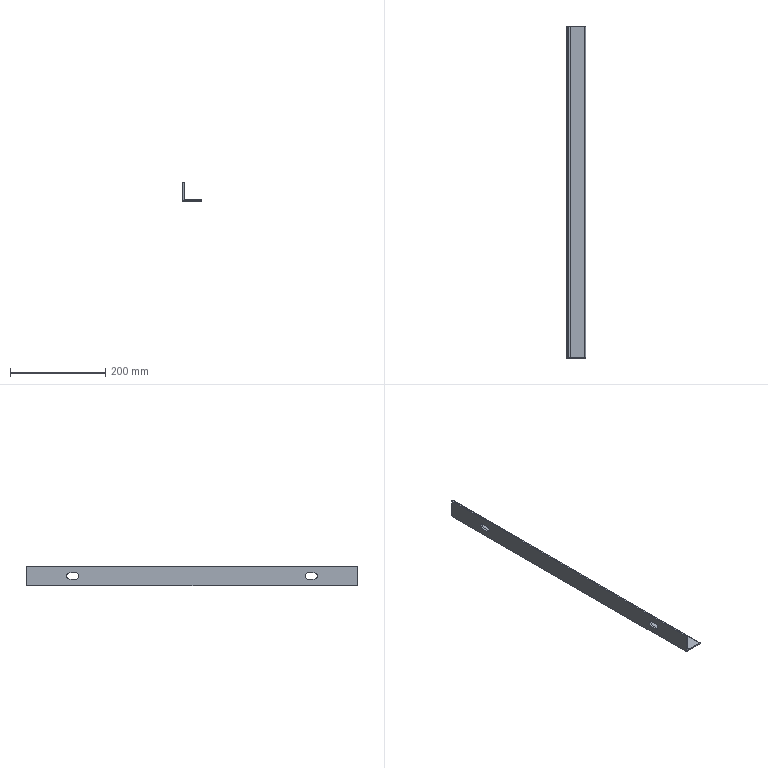Component | SolidWorks | FrameAssembly-1_BeamAngleSteel-1 | 1 solid | 21 faces | box 40 x 696 x 40 mm | volume 210483 mm3 | plane 14 | cylinder 7 | commonest cylinder face diameters 13 x4 2.667 x2 7 x1
build123d program:
from build123d import *

# Parameters (mm, degrees)
BASE_DEPTH         = 696
CUT_EXTRUDE1_DEPTH = 5
CHAMFER1_SIZE      = 1.5


with BuildPart() as part:
    # Sketch1 → Base (new body)
    with BuildSketch(Plane.YZ):
        with BuildLine():
            Line((0, 40), (0, 0))
            Line((0, 0), (40, 0))
            Line((40, 0), (40, 2.667))
            ThreePointArc((40, 2.667), (39.609, 3.609), (38.667, 4))
            Line((38.667, 4), (7.5, 4))
            ThreePointArc((7.5, 4), (5.025, 5.025), (4, 7.5))
            Line((4, 7.5), (4, 38.667))
            ThreePointArc((4, 38.667), (3.609, 39.609), (2.667, 40))
            Line((2.667, 40), (0, 40))
        make_face()
    extrude(amount=BASE_DEPTH)

    # Sketch1_2 → Cut-Extrude1 (cut)
    with BuildSketch(Plane(origin=(0, 4, 0), x_dir=(-1, 0, 0), z_dir=(0, 1, 0))):
        with BuildLine():
            Line((-92, 13.5), (-104, 13.5))
            ThreePointArc((-104, 13.5), (-110.5, 20), (-104, 26.5))
            Line((-104, 26.5), (-92, 26.5))
            ThreePointArc((-92, 26.5), (-85.5, 20), (-92, 13.5))
        make_face()
        with BuildLine():
            Line((-592, 13.5), (-604, 13.5))
            ThreePointArc((-604, 13.5), (-610.5, 20), (-604, 26.5))
            Line((-604, 26.5), (-592, 26.5))
            ThreePointArc((-592, 26.5), (-585.5, 20), (-592, 13.5))
        make_face()
    extrude(amount=-CUT_EXTRUDE1_DEPTH, mode=Mode.SUBTRACT)

    # Chamfer1
    chamfer1_edges = [part.edges().sort_by_distance(p)[0] for p in [
        (696, 20, 0),
        (0, 20, 0),
    ]]
    chamfer(chamfer1_edges, length=CHAMFER1_SIZE)


solid = part.part

# Placed as in the assembly
solid = solid.moved(Location((-927.848, 492.395, 0), (0, 0, -90)))
STEP:
#1=COLOUR_RGB('',0.7922,0.8196,0.9333);
#2=FILL_AREA_STYLE_COLOUR('',#1);
#3=FILL_AREA_STYLE('',(#2));
#4=SURFACE_STYLE_FILL_AREA(#3);
#5=SURFACE_SIDE_STYLE('',(#4));
#6=SURFACE_STYLE_USAGE(.BOTH.,#5);
#7=PRESENTATION_STYLE_ASSIGNMENT((#6));
#8=CARTESIAN_POINT('',(-36.424,19.386,1.575));
#9=VERTEX_POINT('',#8);
#10=CARTESIAN_POINT('',(-36.529,19.386,1.575));
#11=VERTEX_POINT('',#10);
#12=CARTESIAN_POINT('',(-36.529,19.386,1.575));
#13=DIRECTION('',(-1.,0.,0.));
#14=VECTOR('',#13,39.37);
#15=LINE('',#12,#14);
#16=EDGE_CURVE('',#9,#11,#15,.T.);
#17=ORIENTED_EDGE('',*,*,#16,.T.);
#18=CARTESIAN_POINT('',(-36.529,-8.016,1.575));
#19=VERTEX_POINT('',#18);
#20=CARTESIAN_POINT('',(-36.529,-8.016,1.575));
#21=DIRECTION('',(0.,1.,0.));
#22=VECTOR('',#21,39.37);
#23=LINE('',#20,#22);
#24=EDGE_CURVE('',#19,#11,#23,.T.);
#25=ORIENTED_EDGE('',*,*,#24,.F.);
#26=CARTESIAN_POINT('',(-36.424,-8.016,1.575));
#27=VERTEX_POINT('',#26);
#28=CARTESIAN_POINT('',(-36.529,-8.016,1.575));
#29=DIRECTION('',(-1.,0.,0.));
#30=VECTOR('',#29,39.37);
#31=LINE('',#28,#30);
#32=EDGE_CURVE('',#27,#19,#31,.T.);
#33=ORIENTED_EDGE('',*,*,#32,.F.);
#34=CARTESIAN_POINT('',(-36.424,-8.016,1.575));
#35=DIRECTION('',(0.,1.,0.));
#36=VECTOR('',#35,39.37);
#37=LINE('',#34,#36);
#38=EDGE_CURVE('',#27,#9,#37,.T.);
#39=ORIENTED_EDGE('',*,*,#38,.T.);
#40=EDGE_LOOP('',(#17,#25,#33,#39));
#41=FACE_OUTER_BOUND('',#40,.T.);
#42=CARTESIAN_POINT('',(-36.529,-8.016,1.575));
#43=DIRECTION('',(-0.,0.,-1.));
#44=DIRECTION('',(0.,1.,0.));
#45=AXIS2_PLACEMENT_3D('',#42,#43,#44);
#46=PLANE('',#45);
#47=ADVANCED_FACE('',(#41),#46,.F.);
#48=CARTESIAN_POINT('',(-36.529,-4.394,0.5315));
#49=VERTEX_POINT('',#48);
#50=CARTESIAN_POINT('',(-36.529,-3.921,0.5315));
#51=VERTEX_POINT('',#50);
#52=CARTESIAN_POINT('',(-36.529,-8.016,0.5315));
#53=DIRECTION('',(0.,1.,0.));
#54=VECTOR('',#53,39.37);
#55=LINE('',#52,#54);
#56=EDGE_CURVE('',#49,#51,#55,.T.);
#57=ORIENTED_EDGE('',*,*,#56,.T.);
#58=CARTESIAN_POINT('',(-36.529,-3.921,1.043));
#59=VERTEX_POINT('',#58);
#60=CARTESIAN_POINT('',(-36.529,-3.921,0.7874));
#61=DIRECTION('',(1.,-0.,-0.));
#62=DIRECTION('',(0.,-0.,1.));
#63=AXIS2_PLACEMENT_3D('',#60,#61,#62);
#64=CIRCLE('',#63,0.2559);
#65=EDGE_CURVE('',#51,#59,#64,.T.);
#66=ORIENTED_EDGE('',*,*,#65,.T.);
#67=CARTESIAN_POINT('',(-36.529,-4.394,1.043));
#68=VERTEX_POINT('',#67);
#69=CARTESIAN_POINT('',(-36.529,-8.016,1.043));
#70=DIRECTION('',(-0.,-1.,-0.));
#71=VECTOR('',#70,39.37);
#72=LINE('',#69,#71);
#73=EDGE_CURVE('',#59,#68,#72,.T.);
#74=ORIENTED_EDGE('',*,*,#73,.T.);
#75=CARTESIAN_POINT('',(-36.529,-4.394,0.7874));
#76=DIRECTION('',(1.,-0.,-0.));
#77=DIRECTION('',(0.,-0.,1.));
#78=AXIS2_PLACEMENT_3D('',#75,#76,#77);
#79=CIRCLE('',#78,0.2559);
#80=EDGE_CURVE('',#68,#49,#79,.T.);
#81=ORIENTED_EDGE('',*,*,#80,.T.);
#82=EDGE_LOOP('',(#57,#66,#74,#81));
#83=FACE_BOUND('',#82,.T.);
#84=CARTESIAN_POINT('',(-36.529,15.291,0.5315));
#85=VERTEX_POINT('',#84);
#86=CARTESIAN_POINT('',(-36.529,15.764,0.5315));
#87=VERTEX_POINT('',#86);
#88=CARTESIAN_POINT('',(-36.529,-8.016,0.5315));
#89=DIRECTION('',(0.,1.,0.));
#90=VECTOR('',#89,39.37);
#91=LINE('',#88,#90);
#92=EDGE_CURVE('',#85,#87,#91,.T.);
#93=ORIENTED_EDGE('',*,*,#92,.T.);
#94=CARTESIAN_POINT('',(-36.529,15.764,1.043));
#95=VERTEX_POINT('',#94);
#96=CARTESIAN_POINT('',(-36.529,15.764,0.7874));
#97=DIRECTION('',(1.,-0.,-0.));
#98=DIRECTION('',(0.,-0.,1.));
#99=AXIS2_PLACEMENT_3D('',#96,#97,#98);
#100=CIRCLE('',#99,0.2559);
#101=EDGE_CURVE('',#87,#95,#100,.T.);
#102=ORIENTED_EDGE('',*,*,#101,.T.);
#103=CARTESIAN_POINT('',(-36.529,15.291,1.043));
#104=VERTEX_POINT('',#103);
#105=CARTESIAN_POINT('',(-36.529,-8.016,1.043));
#106=DIRECTION('',(-0.,-1.,-0.));
#107=VECTOR('',#106,39.37);
#108=LINE('',#105,#107);
#109=EDGE_CURVE('',#95,#104,#108,.T.);
#110=ORIENTED_EDGE('',*,*,#109,.T.);
#111=CARTESIAN_POINT('',(-36.529,15.291,0.7874));
#112=DIRECTION('',(1.,-0.,-0.));
#113=DIRECTION('',(0.,-0.,1.));
#114=AXIS2_PLACEMENT_3D('',#111,#112,#113);
#115=CIRCLE('',#114,0.2559);
#116=EDGE_CURVE('',#104,#85,#115,.T.);
#117=ORIENTED_EDGE('',*,*,#116,.T.);
#118=EDGE_LOOP('',(#93,#102,#110,#117));
#119=FACE_BOUND('',#118,.T.);
#120=CARTESIAN_POINT('',(-36.529,19.386,0.05906));
#121=VERTEX_POINT('',#120);
#122=CARTESIAN_POINT('',(-36.529,19.386,1.575));
#123=DIRECTION('',(-0.,0.,-1.));
#124=VECTOR('',#123,39.37);
#125=LINE('',#122,#124);
#126=EDGE_CURVE('',#11,#121,#125,.T.);
#127=ORIENTED_EDGE('',*,*,#126,.T.);
#128=CARTESIAN_POINT('',(-36.529,19.327,-0.));
#129=VERTEX_POINT('',#128);
#130=CARTESIAN_POINT('',(-36.529,19.327,-0.));
#131=DIRECTION('',(-0.,-0.7071,-0.7071));
#132=VECTOR('',#131,39.37);
#133=LINE('',#130,#132);
#134=EDGE_CURVE('',#121,#129,#133,.T.);
#135=ORIENTED_EDGE('',*,*,#134,.T.);
#136=CARTESIAN_POINT('',(-36.529,-7.957,-0.));
#137=VERTEX_POINT('',#136);
#138=CARTESIAN_POINT('',(-36.529,-8.016,-0.));
#139=DIRECTION('',(0.,1.,0.));
#140=VECTOR('',#139,39.37);
#141=LINE('',#138,#140);
#142=EDGE_CURVE('',#137,#129,#141,.T.);
#143=ORIENTED_EDGE('',*,*,#142,.F.);
#144=CARTESIAN_POINT('',(-36.529,-8.016,0.05906));
#145=VERTEX_POINT('',#144);
#146=CARTESIAN_POINT('',(-36.529,-8.016,0.05906));
#147=DIRECTION('',(-0.,-0.7071,0.7071));
#148=VECTOR('',#147,39.37);
#149=LINE('',#146,#148);
#150=EDGE_CURVE('',#137,#145,#149,.T.);
#151=ORIENTED_EDGE('',*,*,#150,.T.);
#152=CARTESIAN_POINT('',(-36.529,-8.016,1.575));
#153=DIRECTION('',(-0.,0.,-1.));
#154=VECTOR('',#153,39.37);
#155=LINE('',#152,#154);
#156=EDGE_CURVE('',#19,#145,#155,.T.);
#157=ORIENTED_EDGE('',*,*,#156,.F.);
#158=ORIENTED_EDGE('',*,*,#24,.T.);
#159=EDGE_LOOP('',(#127,#135,#143,#151,#157,#158));
#160=FACE_OUTER_BOUND('',#159,.T.);
#161=CARTESIAN_POINT('',(-36.529,-8.016,1.575));
#162=DIRECTION('',(1.,-0.,-0.));
#163=DIRECTION('',(0.,-0.,1.));
#164=AXIS2_PLACEMENT_3D('',#161,#162,#163);
#165=PLANE('',#164);
#166=ADVANCED_FACE('',(#83,#119,#160),#165,.F.);
#167=ORIENTED_EDGE('',*,*,#142,.T.);
#168=CARTESIAN_POINT('',(-34.955,19.327,-0.));
#169=VERTEX_POINT('',#168);
#170=CARTESIAN_POINT('',(-34.955,19.327,-0.));
#171=DIRECTION('',(1.,-0.,-0.));
#172=VECTOR('',#171,39.37);
#173=LINE('',#170,#172);
#174=EDGE_CURVE('',#129,#169,#173,.T.);
#175=ORIENTED_EDGE('',*,*,#174,.T.);
#176=CARTESIAN_POINT('',(-34.955,-7.957,-0.));
#177=VERTEX_POINT('',#176);
#178=CARTESIAN_POINT('',(-34.955,-8.016,-0.));
#179=DIRECTION('',(0.,1.,0.));
#180=VECTOR('',#179,39.37);
#181=LINE('',#178,#180);
#182=EDGE_CURVE('',#177,#169,#181,.T.);
#183=ORIENTED_EDGE('',*,*,#182,.F.);
#184=CARTESIAN_POINT('',(-36.529,-7.957,-0.));
#185=DIRECTION('',(-1.,0.,0.));
#186=VECTOR('',#185,39.37);
#187=LINE('',#184,#186);
#188=EDGE_CURVE('',#177,#137,#187,.T.);
#189=ORIENTED_EDGE('',*,*,#188,.T.);
#190=EDGE_LOOP('',(#167,#175,#183,#189));
#191=FACE_OUTER_BOUND('',#190,.T.);
#192=CARTESIAN_POINT('',(-36.529,-8.016,-0.));
#193=DIRECTION('',(0.,-0.,1.));
#194=DIRECTION('',(-0.,-1.,-0.));
#195=AXIS2_PLACEMENT_3D('',#192,#193,#194);
#196=PLANE('',#195);
#197=ADVANCED_FACE('',(#191),#196,.F.);
#198=ORIENTED_EDGE('',*,*,#182,.T.);
#199=CARTESIAN_POINT('',(-34.955,19.386,0.05906));
#200=VERTEX_POINT('',#199);
#201=CARTESIAN_POINT('',(-34.955,19.327,-0.));
#202=DIRECTION('',(0.,0.7071,0.7071));
#203=VECTOR('',#202,39.37);
#204=LINE('',#201,#203);
#205=EDGE_CURVE('',#169,#200,#204,.T.);
#206=ORIENTED_EDGE('',*,*,#205,.T.);
#207=CARTESIAN_POINT('',(-34.955,19.386,0.105));
#208=VERTEX_POINT('',#207);
#209=CARTESIAN_POINT('',(-34.955,19.386,-0.));
#210=DIRECTION('',(0.,-0.,1.));
#211=VECTOR('',#210,39.37);
#212=LINE('',#209,#211);
#213=EDGE_CURVE('',#200,#208,#212,.T.);
#214=ORIENTED_EDGE('',*,*,#213,.T.);
#215=CARTESIAN_POINT('',(-34.955,-8.016,0.105));
#216=VERTEX_POINT('',#215);
#217=CARTESIAN_POINT('',(-34.955,-8.016,0.105));
#218=DIRECTION('',(0.,1.,0.));
#219=VECTOR('',#218,39.37);
#220=LINE('',#217,#219);
#221=EDGE_CURVE('',#216,#208,#220,.T.);
#222=ORIENTED_EDGE('',*,*,#221,.F.);
#223=CARTESIAN_POINT('',(-34.955,-8.016,0.05906));
#224=VERTEX_POINT('',#223);
#225=CARTESIAN_POINT('',(-34.955,-8.016,-0.));
#226=DIRECTION('',(0.,-0.,1.));
#227=VECTOR('',#226,39.37);
#228=LINE('',#225,#227);
#229=EDGE_CURVE('',#224,#216,#228,.T.);
#230=ORIENTED_EDGE('',*,*,#229,.F.);
#231=CARTESIAN_POINT('',(-34.955,-8.016,0.05906));
#232=DIRECTION('',(0.,0.7071,-0.7071));
#233=VECTOR('',#232,39.37);
#234=LINE('',#231,#233);
#235=EDGE_CURVE('',#224,#177,#234,.T.);
#236=ORIENTED_EDGE('',*,*,#235,.T.);
#237=EDGE_LOOP('',(#198,#206,#214,#222,#230,#236));
#238=FACE_OUTER_BOUND('',#237,.T.);
#239=CARTESIAN_POINT('',(-34.955,-8.016,-0.));
#240=DIRECTION('',(-1.,0.,0.));
#241=DIRECTION('',(-0.,0.,-1.));
#242=AXIS2_PLACEMENT_3D('',#239,#240,#241);
#243=PLANE('',#242);
#244=ADVANCED_FACE('',(#238),#243,.F.);
#245=CARTESIAN_POINT('',(-35.007,19.386,0.1575));
#246=VERTEX_POINT('',#245);
#247=CARTESIAN_POINT('',(-35.007,19.386,0.105));
#248=DIRECTION('',(-0.,-1.,-0.));
#249=DIRECTION('',(0.,0.,-1.));
#250=AXIS2_PLACEMENT_3D('',#247,#248,#249);
#251=CIRCLE('',#250,0.05249);
#252=EDGE_CURVE('',#208,#246,#251,.T.);
#253=ORIENTED_EDGE('',*,*,#252,.T.);
#254=CARTESIAN_POINT('',(-35.007,-8.016,0.1575));
#255=VERTEX_POINT('',#254);
#256=CARTESIAN_POINT('',(-35.007,-8.016,0.1575));
#257=DIRECTION('',(0.,1.,0.));
#258=VECTOR('',#257,39.37);
#259=LINE('',#256,#258);
#260=EDGE_CURVE('',#255,#246,#259,.T.);
#261=ORIENTED_EDGE('',*,*,#260,.F.);
#262=CARTESIAN_POINT('',(-35.007,-8.016,0.105));
#263=DIRECTION('',(-0.,-1.,-0.));
#264=DIRECTION('',(0.,0.,-1.));
#265=AXIS2_PLACEMENT_3D('',#262,#263,#264);
#266=CIRCLE('',#265,0.05249);
#267=EDGE_CURVE('',#216,#255,#266,.T.);
#268=ORIENTED_EDGE('',*,*,#267,.F.);
#269=ORIENTED_EDGE('',*,*,#221,.T.);
#270=EDGE_LOOP('',(#253,#261,#268,#269));
#271=FACE_OUTER_BOUND('',#270,.T.);
#272=CARTESIAN_POINT('',(-35.007,-8.016,0.105));
#273=DIRECTION('',(0.,1.,0.));
#274=DIRECTION('',(0.,-0.,1.));
#275=AXIS2_PLACEMENT_3D('',#272,#273,#274);
#276=CYLINDRICAL_SURFACE('',#275,0.05249);
#277=ADVANCED_FACE('',(#271),#276,.T.);
#278=CARTESIAN_POINT('',(-36.234,19.386,0.1575));
#279=VERTEX_POINT('',#278);
#280=CARTESIAN_POINT('',(-36.234,19.386,0.1575));
#281=DIRECTION('',(-1.,0.,0.));
#282=VECTOR('',#281,39.37);
#283=LINE('',#280,#282);
#284=EDGE_CURVE('',#246,#279,#283,.T.);
#285=ORIENTED_EDGE('',*,*,#284,.T.);
#286=CARTESIAN_POINT('',(-36.234,-8.016,0.1575));
#287=VERTEX_POINT('',#286);
#288=CARTESIAN_POINT('',(-36.234,-8.016,0.1575));
#289=DIRECTION('',(0.,1.,0.));
#290=VECTOR('',#289,39.37);
#291=LINE('',#288,#290);
#292=EDGE_CURVE('',#287,#279,#291,.T.);
#293=ORIENTED_EDGE('',*,*,#292,.F.);
#294=CARTESIAN_POINT('',(-36.234,-8.016,0.1575));
#295=DIRECTION('',(-1.,0.,0.));
#296=VECTOR('',#295,39.37);
#297=LINE('',#294,#296);
#298=EDGE_CURVE('',#255,#287,#297,.T.);
#299=ORIENTED_EDGE('',*,*,#298,.F.);
#300=ORIENTED_EDGE('',*,*,#260,.T.);
#301=EDGE_LOOP('',(#285,#293,#299,#300));
#302=FACE_OUTER_BOUND('',#301,.T.);
#303=CARTESIAN_POINT('',(-36.234,-8.016,0.1575));
#304=DIRECTION('',(-0.,0.,-1.));
#305=DIRECTION('',(0.,1.,0.));
#306=AXIS2_PLACEMENT_3D('',#303,#304,#305);
#307=PLANE('',#306);
#308=ADVANCED_FACE('',(#302),#307,.F.);
#309=CARTESIAN_POINT('',(-36.372,19.386,0.2953));
#310=VERTEX_POINT('',#309);
#311=CARTESIAN_POINT('',(-36.234,19.386,0.2953));
#312=DIRECTION('',(0.,1.,0.));
#313=DIRECTION('',(0.,0.,-1.));
#314=AXIS2_PLACEMENT_3D('',#311,#312,#313);
#315=CIRCLE('',#314,0.1378);
#316=EDGE_CURVE('',#279,#310,#315,.T.);
#317=ORIENTED_EDGE('',*,*,#316,.T.);
#318=CARTESIAN_POINT('',(-36.372,-8.016,0.2953));
#319=VERTEX_POINT('',#318);
#320=CARTESIAN_POINT('',(-36.372,-8.016,0.2953));
#321=DIRECTION('',(0.,1.,0.));
#322=VECTOR('',#321,39.37);
#323=LINE('',#320,#322);
#324=EDGE_CURVE('',#319,#310,#323,.T.);
#325=ORIENTED_EDGE('',*,*,#324,.F.);
#326=CARTESIAN_POINT('',(-36.234,-8.016,0.2953));
#327=DIRECTION('',(0.,1.,0.));
#328=DIRECTION('',(0.,0.,-1.));
#329=AXIS2_PLACEMENT_3D('',#326,#327,#328);
#330=CIRCLE('',#329,0.1378);
#331=EDGE_CURVE('',#287,#319,#330,.T.);
#332=ORIENTED_EDGE('',*,*,#331,.F.);
#333=ORIENTED_EDGE('',*,*,#292,.T.);
#334=EDGE_LOOP('',(#317,#325,#332,#333));
#335=FACE_OUTER_BOUND('',#334,.T.);
#336=CARTESIAN_POINT('',(-36.234,-8.016,0.2953));
#337=DIRECTION('',(0.,1.,0.));
#338=DIRECTION('',(0.,-0.,1.));
#339=AXIS2_PLACEMENT_3D('',#336,#337,#338);
#340=CYLINDRICAL_SURFACE('',#339,0.1378);
#341=ADVANCED_FACE('',(#335),#340,.F.);
#342=CARTESIAN_POINT('',(-36.372,-3.921,1.043));
#343=VERTEX_POINT('',#342);
#344=CARTESIAN_POINT('',(-36.372,-4.394,1.043));
#345=VERTEX_POINT('',#344);
#346=CARTESIAN_POINT('',(-36.372,-3.921,1.043));
#347=DIRECTION('',(-0.,-1.,-0.));
#348=VECTOR('',#347,39.37);
#349=LINE('',#346,#348);
#350=EDGE_CURVE('',#343,#345,#349,.T.);
#351=ORIENTED_EDGE('',*,*,#350,.F.);
#352=CARTESIAN_POINT('',(-36.372,-3.921,0.5315));
#353=VERTEX_POINT('',#352);
#354=CARTESIAN_POINT('',(-36.372,-3.921,0.7874));
#355=DIRECTION('',(1.,-0.,-0.));
#356=DIRECTION('',(0.,-0.,1.));
#357=AXIS2_PLACEMENT_3D('',#354,#355,#356);
#358=CIRCLE('',#357,0.2559);
#359=EDGE_CURVE('',#353,#343,#358,.T.);
#360=ORIENTED_EDGE('',*,*,#359,.F.);
#361=CARTESIAN_POINT('',(-36.372,-4.394,0.5315));
#362=VERTEX_POINT('',#361);
#363=CARTESIAN_POINT('',(-36.372,-3.921,0.5315));
#364=DIRECTION('',(0.,1.,0.));
#365=VECTOR('',#364,39.37);
#366=LINE('',#363,#365);
#367=EDGE_CURVE('',#362,#353,#366,.T.);
#368=ORIENTED_EDGE('',*,*,#367,.F.);
#369=CARTESIAN_POINT('',(-36.372,-4.394,0.7874));
#370=DIRECTION('',(1.,-0.,-0.));
#371=DIRECTION('',(0.,-0.,1.));
#372=AXIS2_PLACEMENT_3D('',#369,#370,#371);
#373=CIRCLE('',#372,0.2559);
#374=EDGE_CURVE('',#345,#362,#373,.T.);
#375=ORIENTED_EDGE('',*,*,#374,.F.);
#376=EDGE_LOOP('',(#351,#360,#368,#375));
#377=FACE_BOUND('',#376,.T.);
#378=CARTESIAN_POINT('',(-36.372,15.764,1.043));
#379=VERTEX_POINT('',#378);
#380=CARTESIAN_POINT('',(-36.372,15.291,1.043));
#381=VERTEX_POINT('',#380);
#382=CARTESIAN_POINT('',(-36.372,15.764,1.043));
#383=DIRECTION('',(-0.,-1.,-0.));
#384=VECTOR('',#383,39.37);
#385=LINE('',#382,#384);
#386=EDGE_CURVE('',#379,#381,#385,.T.);
#387=ORIENTED_EDGE('',*,*,#386,.F.);
#388=CARTESIAN_POINT('',(-36.372,15.764,0.5315));
#389=VERTEX_POINT('',#388);
#390=CARTESIAN_POINT('',(-36.372,15.764,0.7874));
#391=DIRECTION('',(1.,-0.,-0.));
#392=DIRECTION('',(0.,-0.,1.));
#393=AXIS2_PLACEMENT_3D('',#390,#391,#392);
#394=CIRCLE('',#393,0.2559);
#395=EDGE_CURVE('',#389,#379,#394,.T.);
#396=ORIENTED_EDGE('',*,*,#395,.F.);
#397=CARTESIAN_POINT('',(-36.372,15.291,0.5315));
#398=VERTEX_POINT('',#397);
#399=CARTESIAN_POINT('',(-36.372,15.764,0.5315));
#400=DIRECTION('',(0.,1.,0.));
#401=VECTOR('',#400,39.37);
#402=LINE('',#399,#401);
#403=EDGE_CURVE('',#398,#389,#402,.T.);
#404=ORIENTED_EDGE('',*,*,#403,.F.);
#405=CARTESIAN_POINT('',(-36.372,15.291,0.7874));
#406=DIRECTION('',(1.,-0.,-0.));
#407=DIRECTION('',(0.,-0.,1.));
#408=AXIS2_PLACEMENT_3D('',#405,#406,#407);
#409=CIRCLE('',#408,0.2559);
#410=EDGE_CURVE('',#381,#398,#409,.T.);
#411=ORIENTED_EDGE('',*,*,#410,.F.);
#412=EDGE_LOOP('',(#387,#396,#404,#411));
#413=FACE_BOUND('',#412,.T.);
#414=CARTESIAN_POINT('',(-36.372,19.386,1.522));
#415=VERTEX_POINT('',#414);
#416=CARTESIAN_POINT('',(-36.372,19.386,1.522));
#417=DIRECTION('',(0.,-0.,1.));
#418=VECTOR('',#417,39.37);
#419=LINE('',#416,#418);
#420=EDGE_CURVE('',#310,#415,#419,.T.);
#421=ORIENTED_EDGE('',*,*,#420,.T.);
#422=CARTESIAN_POINT('',(-36.372,-8.016,1.522));
#423=VERTEX_POINT('',#422);
#424=CARTESIAN_POINT('',(-36.372,-8.016,1.522));
#425=DIRECTION('',(0.,1.,0.));
#426=VECTOR('',#425,39.37);
#427=LINE('',#424,#426);
#428=EDGE_CURVE('',#423,#415,#427,.T.);
#429=ORIENTED_EDGE('',*,*,#428,.F.);
#430=CARTESIAN_POINT('',(-36.372,-8.016,1.522));
#431=DIRECTION('',(0.,-0.,1.));
#432=VECTOR('',#431,39.37);
#433=LINE('',#430,#432);
#434=EDGE_CURVE('',#319,#423,#433,.T.);
#435=ORIENTED_EDGE('',*,*,#434,.F.);
#436=ORIENTED_EDGE('',*,*,#324,.T.);
#437=EDGE_LOOP('',(#421,#429,#435,#436));
#438=FACE_OUTER_BOUND('',#437,.T.);
#439=CARTESIAN_POINT('',(-36.372,-8.016,1.522));
#440=DIRECTION('',(-1.,0.,0.));
#441=DIRECTION('',(-0.,0.,-1.));
#442=AXIS2_PLACEMENT_3D('',#439,#440,#441);
#443=PLANE('',#442);
#444=ADVANCED_FACE('',(#377,#413,#438),#443,.F.);
#445=CARTESIAN_POINT('',(-36.424,19.386,1.522));
#446=DIRECTION('',(-0.,-1.,-0.));
#447=DIRECTION('',(0.,0.,1.));
#448=AXIS2_PLACEMENT_3D('',#445,#446,#447);
#449=CIRCLE('',#448,0.05249);
#450=EDGE_CURVE('',#415,#9,#449,.T.);
#451=ORIENTED_EDGE('',*,*,#450,.T.);
#452=ORIENTED_EDGE('',*,*,#38,.F.);
#453=CARTESIAN_POINT('',(-36.424,-8.016,1.522));
#454=DIRECTION('',(-0.,-1.,-0.));
#455=DIRECTION('',(0.,-0.,1.));
#456=AXIS2_PLACEMENT_3D('',#453,#454,#455);
#457=CIRCLE('',#456,0.05249);
#458=EDGE_CURVE('',#423,#27,#457,.T.);
#459=ORIENTED_EDGE('',*,*,#458,.F.);
#460=ORIENTED_EDGE('',*,*,#428,.T.);
#461=EDGE_LOOP('',(#451,#452,#459,#460));
#462=FACE_OUTER_BOUND('',#461,.T.);
#463=CARTESIAN_POINT('',(-36.424,-8.016,1.522));
#464=DIRECTION('',(0.,1.,0.));
#465=DIRECTION('',(0.,-0.,1.));
#466=AXIS2_PLACEMENT_3D('',#463,#464,#465);
#467=CYLINDRICAL_SURFACE('',#466,0.05249);
#468=ADVANCED_FACE('',(#462),#467,.T.);
#469=ORIENTED_EDGE('',*,*,#156,.T.);
#470=CARTESIAN_POINT('',(-36.424,-8.016,0.05906));
#471=DIRECTION('',(1.,-0.,-0.));
#472=VECTOR('',#471,39.37);
#473=LINE('',#470,#472);
#474=EDGE_CURVE('',#145,#224,#473,.T.);
#475=ORIENTED_EDGE('',*,*,#474,.T.);
#476=ORIENTED_EDGE('',*,*,#229,.T.);
#477=ORIENTED_EDGE('',*,*,#267,.T.);
#478=ORIENTED_EDGE('',*,*,#298,.T.);
#479=ORIENTED_EDGE('',*,*,#331,.T.);
#480=ORIENTED_EDGE('',*,*,#434,.T.);
#481=ORIENTED_EDGE('',*,*,#458,.T.);
#482=ORIENTED_EDGE('',*,*,#32,.T.);
#483=EDGE_LOOP('',(#469,#475,#476,#477,#478,#479,#480,#481,#482));
#484=FACE_OUTER_BOUND('',#483,.T.);
#485=CARTESIAN_POINT('',(-36.424,-8.016,1.522));
#486=DIRECTION('',(0.,1.,0.));
#487=DIRECTION('',(0.,-0.,1.));
#488=AXIS2_PLACEMENT_3D('',#485,#486,#487);
#489=PLANE('',#488);
#490=ADVANCED_FACE('',(#484),#489,.F.);
#491=ORIENTED_EDGE('',*,*,#213,.F.);
#492=CARTESIAN_POINT('',(-36.529,19.386,0.05906));
#493=DIRECTION('',(-1.,0.,0.));
#494=VECTOR('',#493,39.37);
#495=LINE('',#492,#494);
#496=EDGE_CURVE('',#200,#121,#495,.T.);
#497=ORIENTED_EDGE('',*,*,#496,.T.);
#498=ORIENTED_EDGE('',*,*,#126,.F.);
#499=ORIENTED_EDGE('',*,*,#16,.F.);
#500=ORIENTED_EDGE('',*,*,#450,.F.);
#501=ORIENTED_EDGE('',*,*,#420,.F.);
#502=ORIENTED_EDGE('',*,*,#316,.F.);
#503=ORIENTED_EDGE('',*,*,#284,.F.);
#504=ORIENTED_EDGE('',*,*,#252,.F.);
#505=EDGE_LOOP('',(#491,#497,#498,#499,#500,#501,#502,#503,#504));
#506=FACE_OUTER_BOUND('',#505,.T.);
#507=CARTESIAN_POINT('',(-36.424,19.386,1.522));
#508=DIRECTION('',(0.,1.,0.));
#509=DIRECTION('',(0.,-0.,1.));
#510=AXIS2_PLACEMENT_3D('',#507,#508,#509);
#511=PLANE('',#510);
#512=ADVANCED_FACE('',(#506),#511,.T.);
#513=CARTESIAN_POINT('',(-36.569,15.764,0.5315));
#514=DIRECTION('',(1.,-0.,-0.));
#515=VECTOR('',#514,39.37);
#516=LINE('',#513,#515);
#517=EDGE_CURVE('',#87,#389,#516,.T.);
#518=ORIENTED_EDGE('',*,*,#517,.T.);
#519=ORIENTED_EDGE('',*,*,#395,.T.);
#520=CARTESIAN_POINT('',(-36.569,15.764,1.043));
#521=DIRECTION('',(1.,-0.,-0.));
#522=VECTOR('',#521,39.37);
#523=LINE('',#520,#522);
#524=EDGE_CURVE('',#95,#379,#523,.T.);
#525=ORIENTED_EDGE('',*,*,#524,.F.);
#526=ORIENTED_EDGE('',*,*,#101,.F.);
#527=EDGE_LOOP('',(#518,#519,#525,#526));
#528=FACE_OUTER_BOUND('',#527,.T.);
#529=CARTESIAN_POINT('',(-36.569,15.764,0.7874));
#530=DIRECTION('',(1.,-0.,-0.));
#531=DIRECTION('',(0.,-0.,1.));
#532=AXIS2_PLACEMENT_3D('',#529,#530,#531);
#533=CYLINDRICAL_SURFACE('',#532,0.2559);
#534=ADVANCED_FACE('',(#528),#533,.F.);
#535=CARTESIAN_POINT('',(-36.569,15.291,0.5315));
#536=DIRECTION('',(1.,-0.,-0.));
#537=VECTOR('',#536,39.37);
#538=LINE('',#535,#537);
#539=EDGE_CURVE('',#85,#398,#538,.T.);
#540=ORIENTED_EDGE('',*,*,#539,.T.);
#541=ORIENTED_EDGE('',*,*,#403,.T.);
#542=ORIENTED_EDGE('',*,*,#517,.F.);
#543=ORIENTED_EDGE('',*,*,#92,.F.);
#544=EDGE_LOOP('',(#540,#541,#542,#543));
#545=FACE_OUTER_BOUND('',#544,.T.);
#546=CARTESIAN_POINT('',(-36.569,15.764,0.5315));
#547=DIRECTION('',(-0.,0.,-1.));
#548=DIRECTION('',(0.,1.,0.));
#549=AXIS2_PLACEMENT_3D('',#546,#547,#548);
#550=PLANE('',#549);
#551=ADVANCED_FACE('',(#545),#550,.F.);
#552=CARTESIAN_POINT('',(-36.569,15.291,1.043));
#553=DIRECTION('',(1.,-0.,-0.));
#554=VECTOR('',#553,39.37);
#555=LINE('',#552,#554);
#556=EDGE_CURVE('',#104,#381,#555,.T.);
#557=ORIENTED_EDGE('',*,*,#556,.T.);
#558=ORIENTED_EDGE('',*,*,#410,.T.);
#559=ORIENTED_EDGE('',*,*,#539,.F.);
#560=ORIENTED_EDGE('',*,*,#116,.F.);
#561=EDGE_LOOP('',(#557,#558,#559,#560));
#562=FACE_OUTER_BOUND('',#561,.T.);
#563=CARTESIAN_POINT('',(-36.569,15.291,0.7874));
#564=DIRECTION('',(1.,-0.,-0.));
#565=DIRECTION('',(0.,-0.,1.));
#566=AXIS2_PLACEMENT_3D('',#563,#564,#565);
#567=CYLINDRICAL_SURFACE('',#566,0.2559);
#568=ADVANCED_FACE('',(#562),#567,.F.);
#569=ORIENTED_EDGE('',*,*,#524,.T.);
#570=ORIENTED_EDGE('',*,*,#386,.T.);
#571=ORIENTED_EDGE('',*,*,#556,.F.);
#572=ORIENTED_EDGE('',*,*,#109,.F.);
#573=EDGE_LOOP('',(#569,#570,#571,#572));
#574=FACE_OUTER_BOUND('',#573,.T.);
#575=CARTESIAN_POINT('',(-36.569,15.764,1.043));
#576=DIRECTION('',(0.,-0.,1.));
#577=DIRECTION('',(-1.,0.,0.));
#578=AXIS2_PLACEMENT_3D('',#575,#576,#577);
#579=PLANE('',#578);
#580=ADVANCED_FACE('',(#574),#579,.F.);
#581=CARTESIAN_POINT('',(-36.569,-3.921,0.5315));
#582=DIRECTION('',(1.,-0.,-0.));
#583=VECTOR('',#582,39.37);
#584=LINE('',#581,#583);
#585=EDGE_CURVE('',#51,#353,#584,.T.);
#586=ORIENTED_EDGE('',*,*,#585,.T.);
#587=ORIENTED_EDGE('',*,*,#359,.T.);
#588=CARTESIAN_POINT('',(-36.569,-3.921,1.043));
#589=DIRECTION('',(1.,-0.,-0.));
#590=VECTOR('',#589,39.37);
#591=LINE('',#588,#590);
#592=EDGE_CURVE('',#59,#343,#591,.T.);
#593=ORIENTED_EDGE('',*,*,#592,.F.);
#594=ORIENTED_EDGE('',*,*,#65,.F.);
#595=EDGE_LOOP('',(#586,#587,#593,#594));
#596=FACE_OUTER_BOUND('',#595,.T.);
#597=CARTESIAN_POINT('',(-36.569,-3.921,0.7874));
#598=DIRECTION('',(1.,-0.,-0.));
#599=DIRECTION('',(0.,-0.,1.));
#600=AXIS2_PLACEMENT_3D('',#597,#598,#599);
#601=CYLINDRICAL_SURFACE('',#600,0.2559);
#602=ADVANCED_FACE('',(#596),#601,.F.);
#603=CARTESIAN_POINT('',(-36.569,-4.394,0.5315));
#604=DIRECTION('',(1.,-0.,-0.));
#605=VECTOR('',#604,39.37);
#606=LINE('',#603,#605);
#607=EDGE_CURVE('',#49,#362,#606,.T.);
#608=ORIENTED_EDGE('',*,*,#607,.T.);
#609=ORIENTED_EDGE('',*,*,#367,.T.);
#610=ORIENTED_EDGE('',*,*,#585,.F.);
#611=ORIENTED_EDGE('',*,*,#56,.F.);
#612=EDGE_LOOP('',(#608,#609,#610,#611));
#613=FACE_OUTER_BOUND('',#612,.T.);
#614=CARTESIAN_POINT('',(-36.569,-3.921,0.5315));
#615=DIRECTION('',(-0.,0.,-1.));
#616=DIRECTION('',(0.,1.,0.));
#617=AXIS2_PLACEMENT_3D('',#614,#615,#616);
#618=PLANE('',#617);
#619=ADVANCED_FACE('',(#613),#618,.F.);
#620=CARTESIAN_POINT('',(-36.569,-4.394,1.043));
#621=DIRECTION('',(1.,-0.,-0.));
#622=VECTOR('',#621,39.37);
#623=LINE('',#620,#622);
#624=EDGE_CURVE('',#68,#345,#623,.T.);
#625=ORIENTED_EDGE('',*,*,#624,.T.);
#626=ORIENTED_EDGE('',*,*,#374,.T.);
#627=ORIENTED_EDGE('',*,*,#607,.F.);
#628=ORIENTED_EDGE('',*,*,#80,.F.);
#629=EDGE_LOOP('',(#625,#626,#627,#628));
#630=FACE_OUTER_BOUND('',#629,.T.);
#631=CARTESIAN_POINT('',(-36.569,-4.394,0.7874));
#632=DIRECTION('',(1.,-0.,-0.));
#633=DIRECTION('',(0.,-0.,1.));
#634=AXIS2_PLACEMENT_3D('',#631,#632,#633);
#635=CYLINDRICAL_SURFACE('',#634,0.2559);
#636=ADVANCED_FACE('',(#630),#635,.F.);
#637=ORIENTED_EDGE('',*,*,#592,.T.);
#638=ORIENTED_EDGE('',*,*,#350,.T.);
#639=ORIENTED_EDGE('',*,*,#624,.F.);
#640=ORIENTED_EDGE('',*,*,#73,.F.);
#641=EDGE_LOOP('',(#637,#638,#639,#640));
#642=FACE_OUTER_BOUND('',#641,.T.);
#643=CARTESIAN_POINT('',(-36.569,-3.921,1.043));
#644=DIRECTION('',(0.,-0.,1.));
#645=DIRECTION('',(-1.,0.,0.));
#646=AXIS2_PLACEMENT_3D('',#643,#644,#645);
#647=PLANE('',#646);
#648=ADVANCED_FACE('',(#642),#647,.F.);
#649=ORIENTED_EDGE('',*,*,#134,.F.);
#650=ORIENTED_EDGE('',*,*,#496,.F.);
#651=ORIENTED_EDGE('',*,*,#205,.F.);
#652=ORIENTED_EDGE('',*,*,#174,.F.);
#653=EDGE_LOOP('',(#649,#650,#651,#652));
#654=FACE_OUTER_BOUND('',#653,.T.);
#655=CARTESIAN_POINT('',(-36.529,19.327,-0.));
#656=DIRECTION('',(0.,0.7071,-0.7071));
#657=DIRECTION('',(-1.,0.,0.));
#658=AXIS2_PLACEMENT_3D('',#655,#656,#657);
#659=PLANE('',#658);
#660=ADVANCED_FACE('',(#654),#659,.T.);
#661=ORIENTED_EDGE('',*,*,#150,.F.);
#662=ORIENTED_EDGE('',*,*,#188,.F.);
#663=ORIENTED_EDGE('',*,*,#235,.F.);
#664=ORIENTED_EDGE('',*,*,#474,.F.);
#665=EDGE_LOOP('',(#661,#662,#663,#664));
#666=FACE_OUTER_BOUND('',#665,.T.);
#667=CARTESIAN_POINT('',(-36.424,-8.016,0.05906));
#668=DIRECTION('',(0.,0.7071,0.7071));
#669=DIRECTION('',(1.,-0.,-0.));
#670=AXIS2_PLACEMENT_3D('',#667,#668,#669);
#671=PLANE('',#670);
#672=ADVANCED_FACE('',(#666),#671,.F.);
#673=CLOSED_SHELL('',(#47,#166,#197,#244,#277,#308,#341,#444,#468,#490,#512,#534,#551,#568,#580,#602,#619,#636,#648,#660,#672));
#674=MANIFOLD_SOLID_BREP('',#673);
#675=STYLED_ITEM('',(#7),#674);
#676=PRESENTATION_LAYER_ASSIGNMENT('','',(#675));
#677=CARTESIAN_POINT('',(0.,0.,0.));
#678=DIRECTION('',(0.,0.,1.));
#679=DIRECTION('',(1.,0.,0.));
#680=AXIS2_PLACEMENT_3D('',#677,#678,#679);
#681=(LENGTH_UNIT()NAMED_UNIT(*)SI_UNIT($,.METRE.));
#682=LENGTH_MEASURE_WITH_UNIT(LENGTH_MEASURE(0.0254),#681);
#683=DIMENSIONAL_EXPONENTS(1.,0.,0.,0.,0.,0.,0.);
#684=(CONVERSION_BASED_UNIT('',#682)LENGTH_UNIT()NAMED_UNIT(#683));
#685=UNCERTAINTY_MEASURE_WITH_UNIT(LENGTH_MEASURE(0.00001),#684,'','');
#686=(NAMED_UNIT(*)PLANE_ANGLE_UNIT()SI_UNIT($,.RADIAN.));
#687=(NAMED_UNIT(*)SI_UNIT($,.STERADIAN.)SOLID_ANGLE_UNIT());
#688=(GEOMETRIC_REPRESENTATION_CONTEXT(3)GLOBAL_UNCERTAINTY_ASSIGNED_CONTEXT((#685))GLOBAL_UNIT_ASSIGNED_CONTEXT((#684,#686,#687))REPRESENTATION_CONTEXT('',''));
#689=ADVANCED_BREP_SHAPE_REPRESENTATION('',(#674,#680),#688);
#690=(LENGTH_UNIT()NAMED_UNIT(*)SI_UNIT($,.METRE.));
#691=LENGTH_MEASURE_WITH_UNIT(LENGTH_MEASURE(0.0254),#690);
#692=DIMENSIONAL_EXPONENTS(1.,0.,0.,0.,0.,0.,0.);
#693=(CONVERSION_BASED_UNIT('',#691)LENGTH_UNIT()NAMED_UNIT(#692));
#694=UNCERTAINTY_MEASURE_WITH_UNIT(LENGTH_MEASURE(0.00001),#693,'','');
#695=(NAMED_UNIT(*)PLANE_ANGLE_UNIT()SI_UNIT($,.RADIAN.));
#696=(NAMED_UNIT(*)SI_UNIT($,.STERADIAN.)SOLID_ANGLE_UNIT());
#697=(GEOMETRIC_REPRESENTATION_CONTEXT(3)GLOBAL_UNCERTAINTY_ASSIGNED_CONTEXT((#694))GLOBAL_UNIT_ASSIGNED_CONTEXT((#693,#695,#696))REPRESENTATION_CONTEXT('',''));
#698=MECHANICAL_DESIGN_GEOMETRIC_PRESENTATION_REPRESENTATION('',(#675),#697);